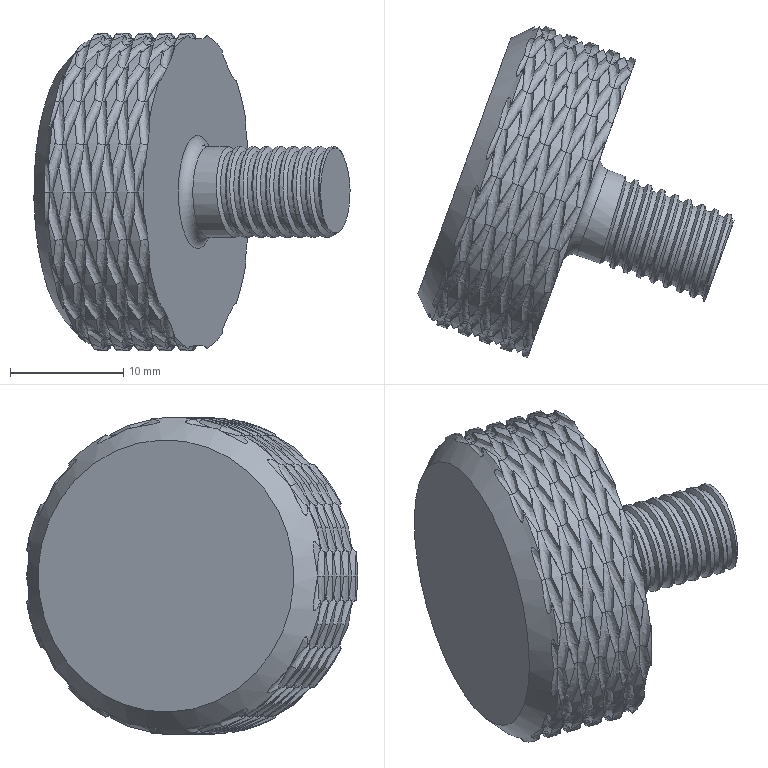Component | NX | 7 | 1 solid | 317 faces | volume 6974 mm3 | spline 202 | cylinder 109 | plane 4 | cone 1 | torus 1 | commonest cylinder face diameters 28 x100 8 x8 7.18 x1